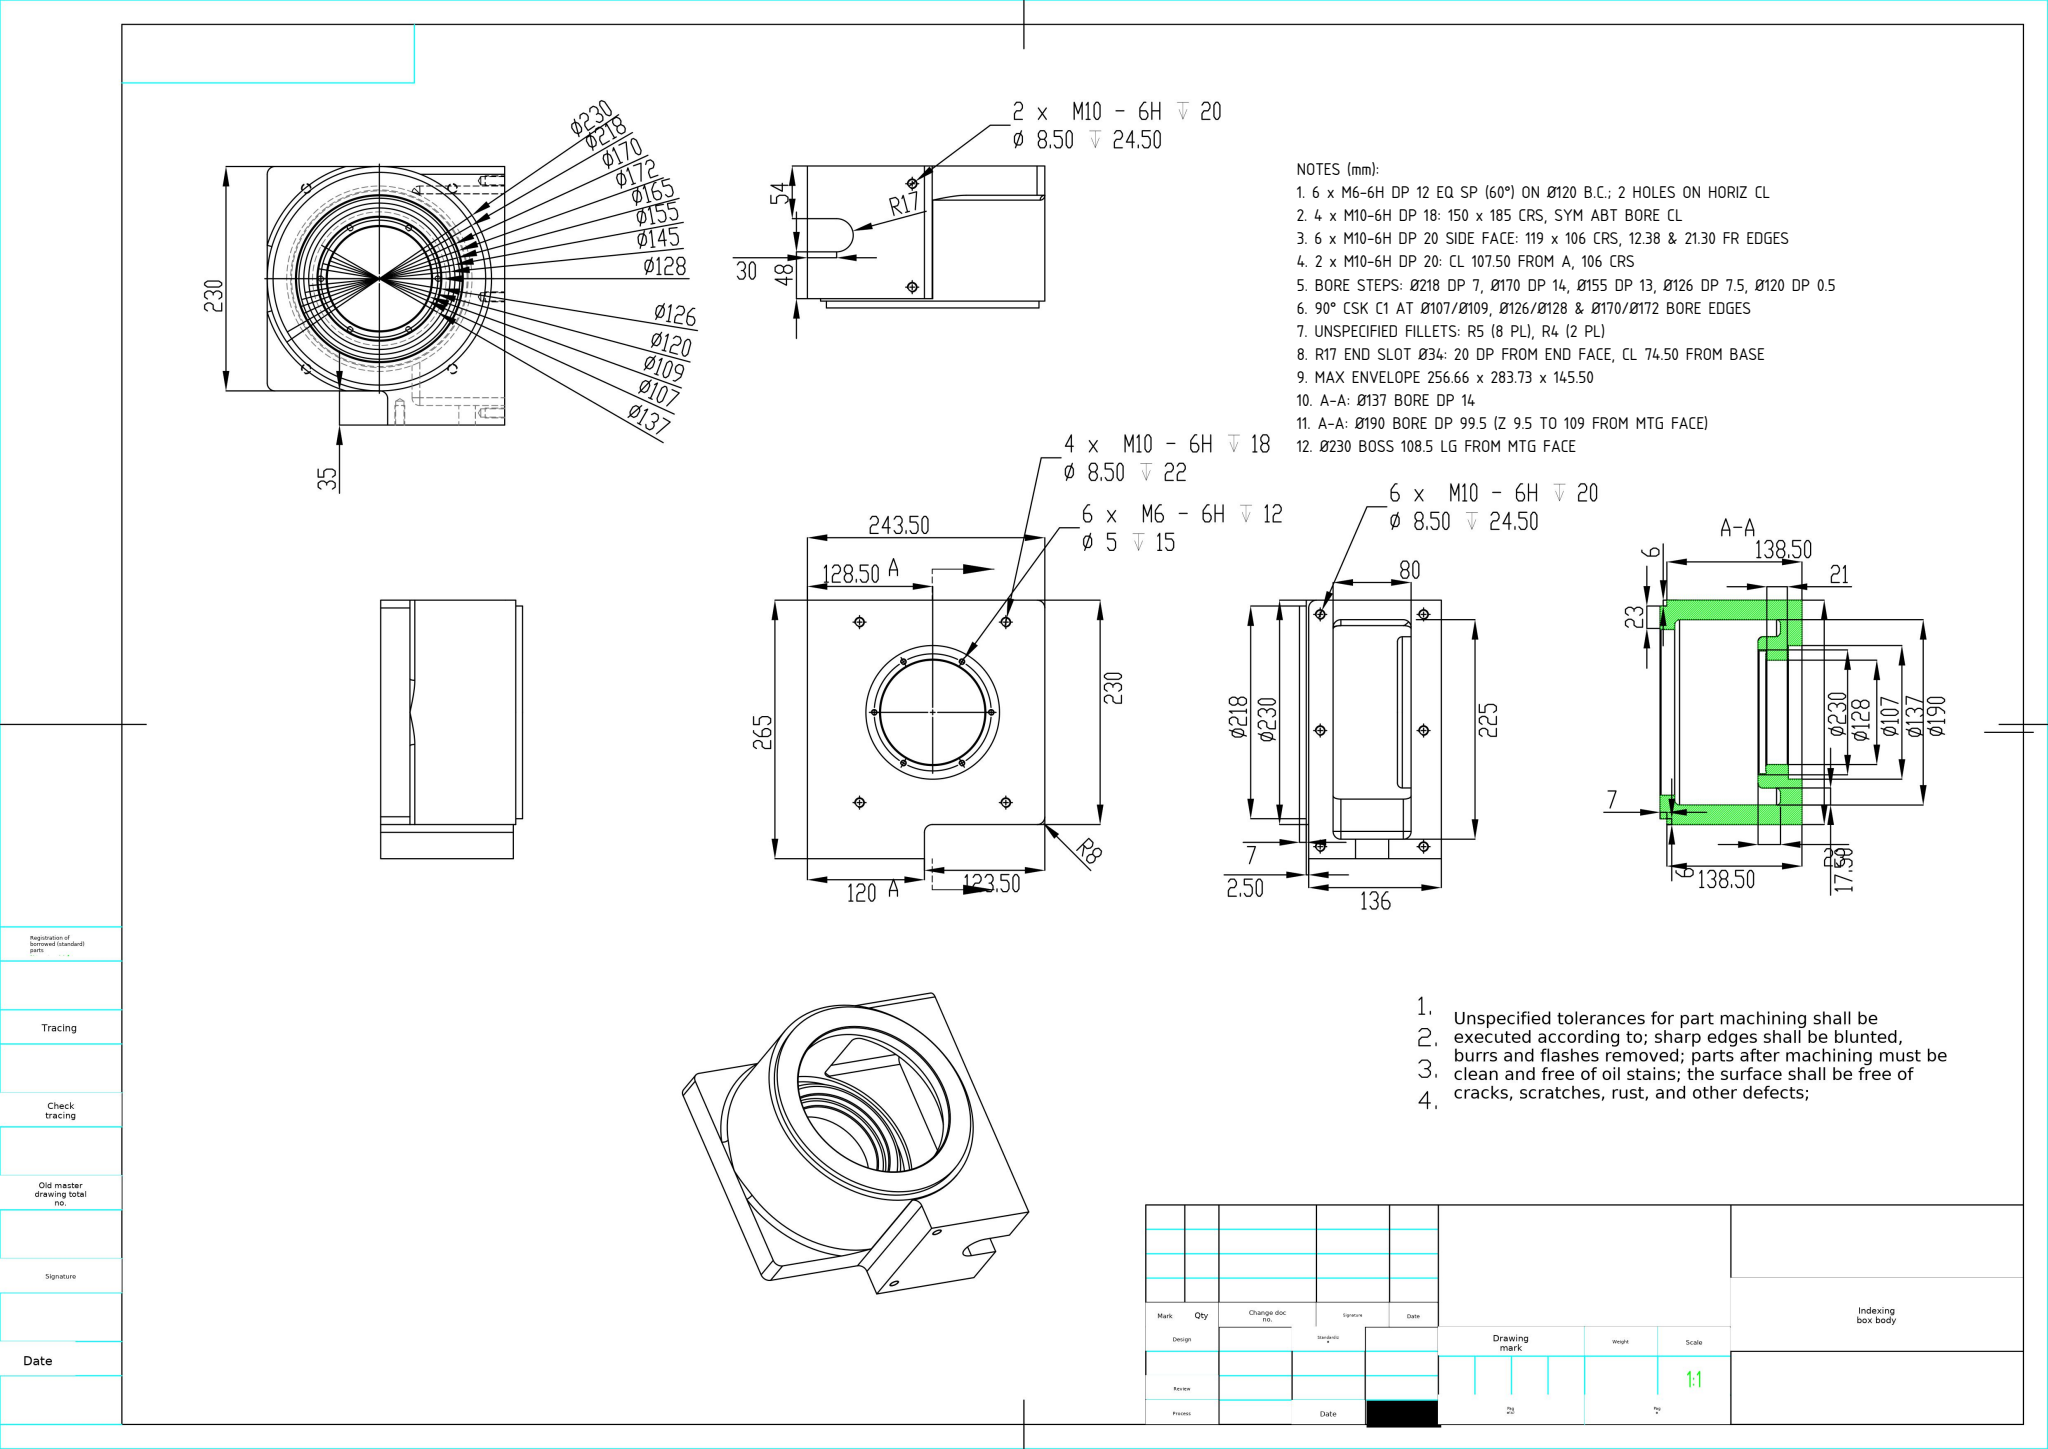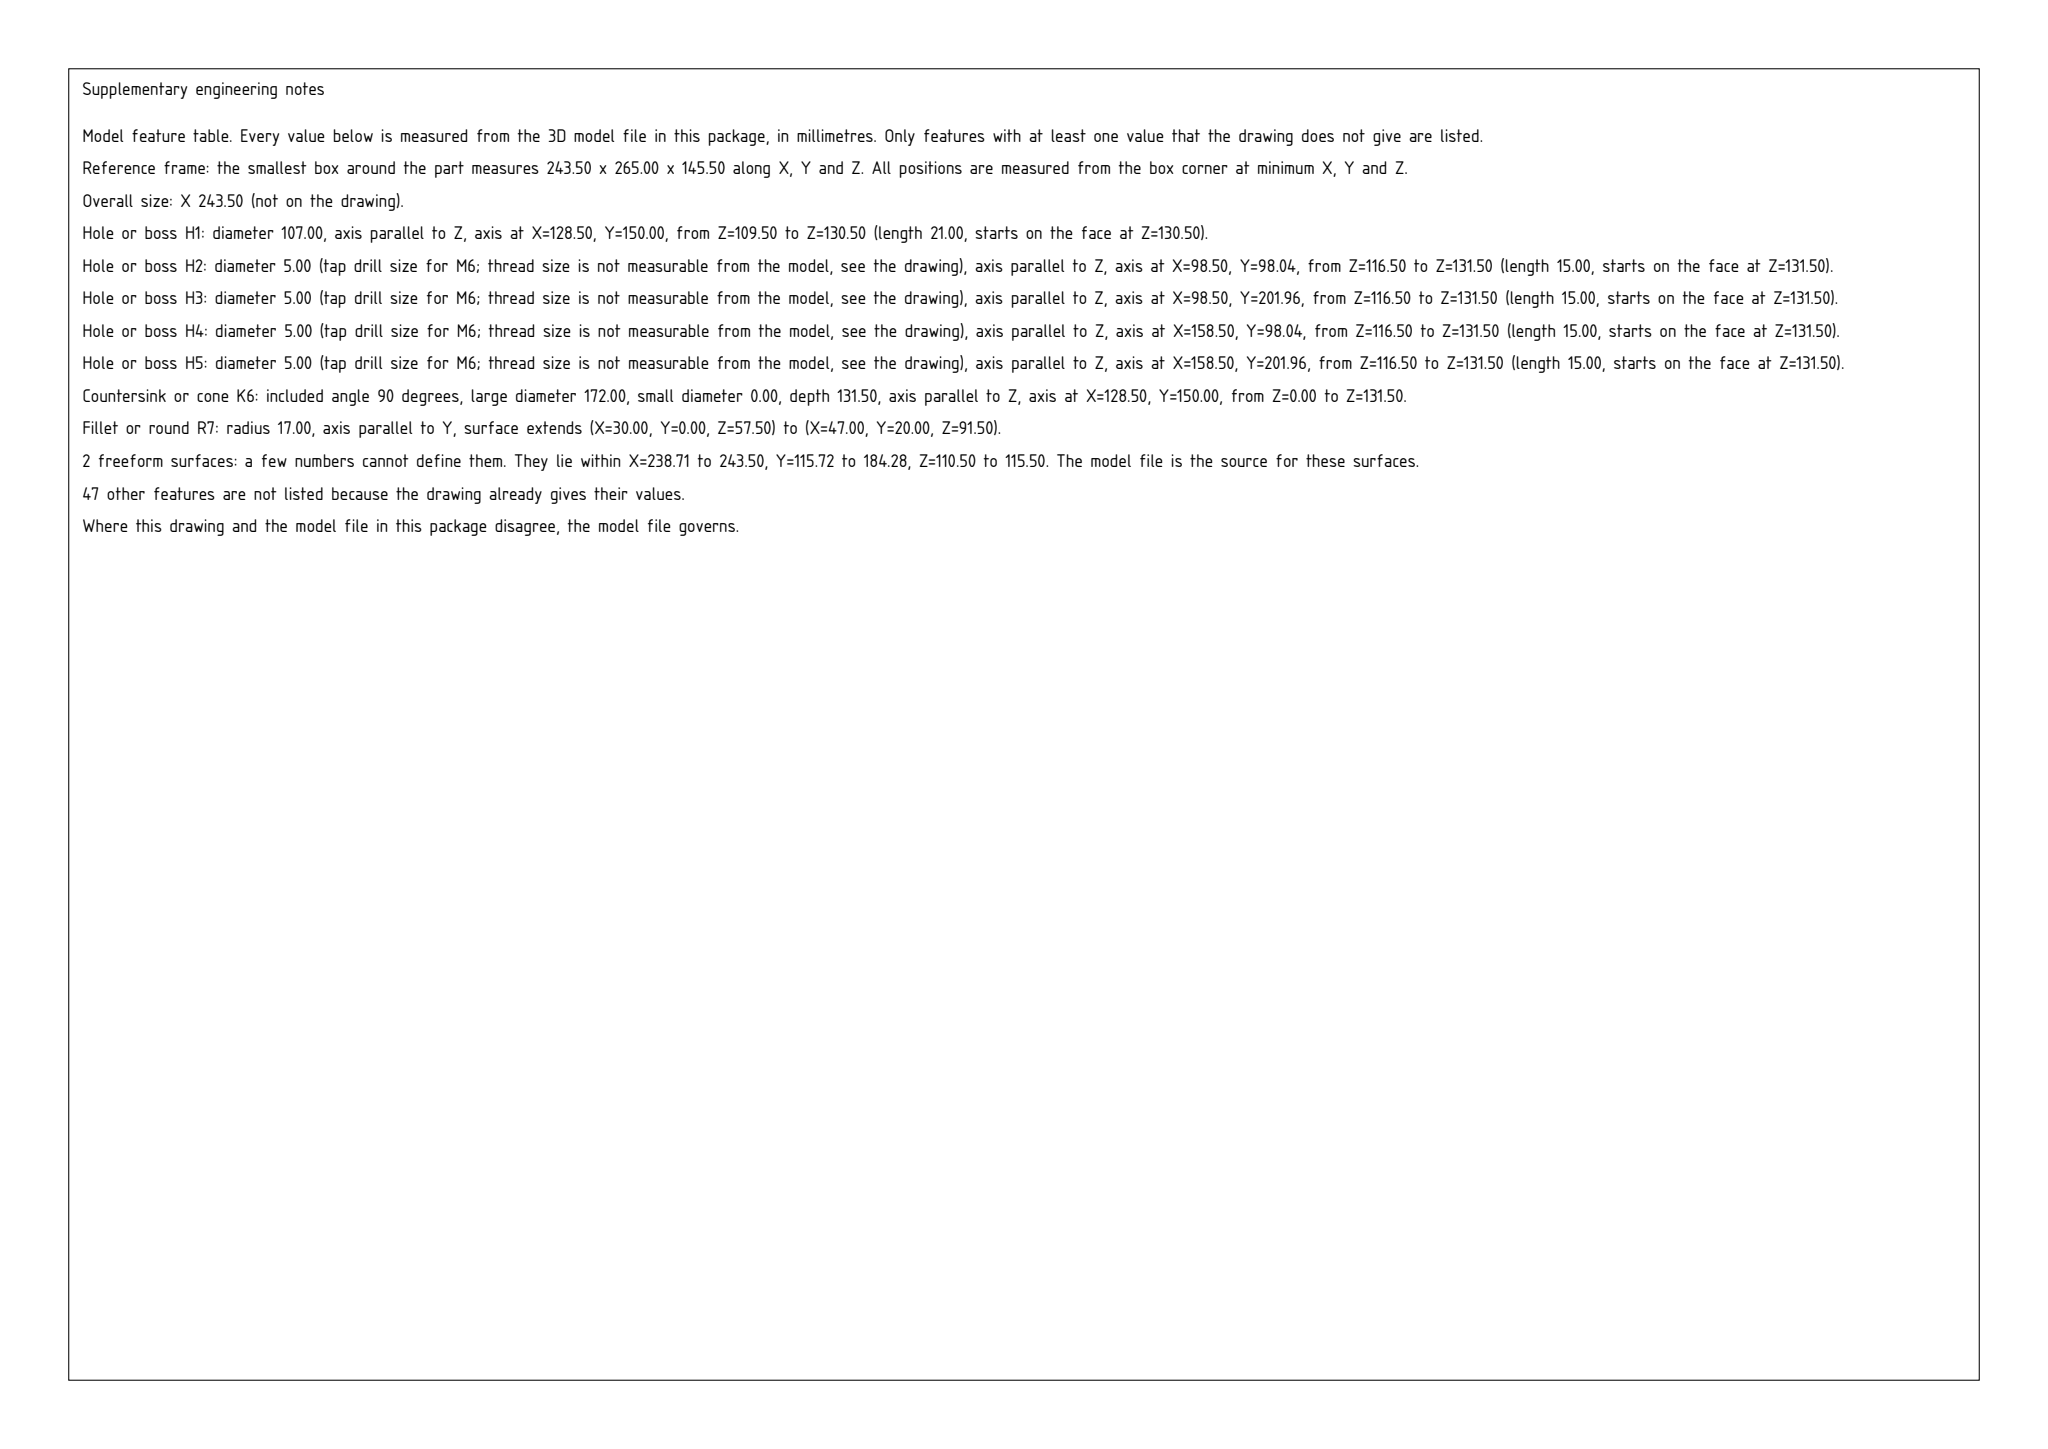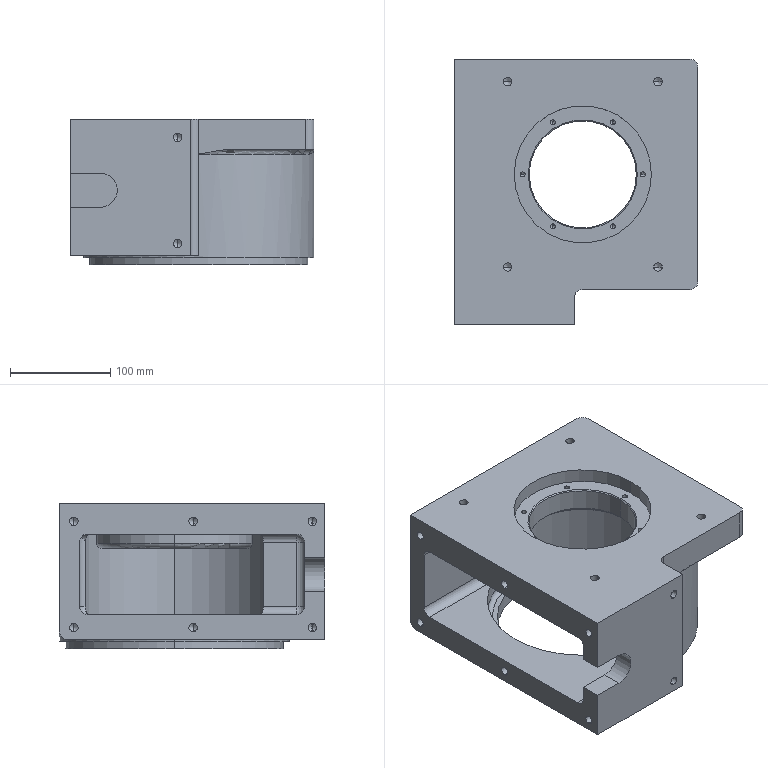Part | SolidWorks | mm | 1 solid | 153 faces | box 243.5 x 265 x 145.5 mm | volume 3346641 mm3 | cylinder 69 | cone 44 | plane 25 | torus 10 | sphere 3 | spline 2 | commonest cylinder face diameters 8.5 x24 16 x14 5 x12 137 x2 107 x2 120 x2 126 x2 155 x2
Drawing notes:
6 x M6-6H DP 12 EQ SP (60°) ON Ø120 B.C.; 2 HOLES ON HORIZ CL | from the solid: Ø5↧15 holes at (68.5,150)(98.5,98.04)(98.5,201.96)(158.5,98.04)(158.5,201.96)(188.5,150) abt ctr (128.5,150) = R60, 60° spacing
4 x M10-6H DP 18: 150 x 185 CRS, SYM ABT BORE CL | from the solid: Ø8.5↧22 z-holes at (53.5,57.5)(53.5,242.5)(203.5,57.5)(203.5,242.5); 203.5-53.5=150, 242.5-57.5=185, ctr=(128.5,150)
6 x M10-6H DP 20 SIDE FACE: 119 x 106 CRS, 12.38 & 21.30 FR EDGES | from the solid: Ø8.5 x-axis holes at y=12.38/131.38/250.38 (pitch 119), z=21.3/127.3 (pitch 106)
2 x M10-6H DP 20: CL 107.50 FROM A, 106 CRS | from the solid: Ø8.5↧24.5 y-axis holes at x=107.5, z=21.3 & 127.3 (106 apart)
BORE STEPS: Ø218 DP 7, Ø170 DP 14, Ø155 DP 13, Ø126 DP 7.5, Ø120 DP 0.5 | from the solid: z-cyl lengths: Ø218=7.0, Ø170=14.0, Ø155=13.0, Ø126=7.5, Ø120=0.5
90° CSK C1 AT Ø107/Ø109, Ø126/Ø128 & Ø170/Ø172 BORE EDGES | from the solid: cones 90° incl, ref dia 107,109,126,172; radial step 1.0 each -> C1
UNSPECIFIED FILLETS: R5 (8 PL), R4 (2 PL) | from the solid: fillet_radii [[4.0,2],[5.0,8]]
R17 END SLOT Ø34: 20 DP FROM END FACE, CL 74.50 FROM BASE | from the solid: Ø34 y-axis cyl, len 20 between y-planes 0 & 20, at x=30.0, z=74.5
MAX ENVELOPE 256.66 x 283.73 x 145.50 | from the solid: bbox_xyz [256.658, 283.73, 145.5]
A-A: Ø137 BORE DP 14 | from the solid: cylinder [137.0,'z',[128.5,150.0],length 14.0]
A-A: Ø190 BORE DP 99.5 (Z 9.5 TO 109 FROM MTG FACE) | from the solid: cylinder [190.0,'z',[128.5,150.0],length 99.5]; z-planes 9.5 and 109.0
Ø230 BOSS 108.5 LG FROM MTG FACE | from the solid: cylinder [230.0,'z',[128.5,150.0],length 108.5]; z-planes 0.0 and 108.5